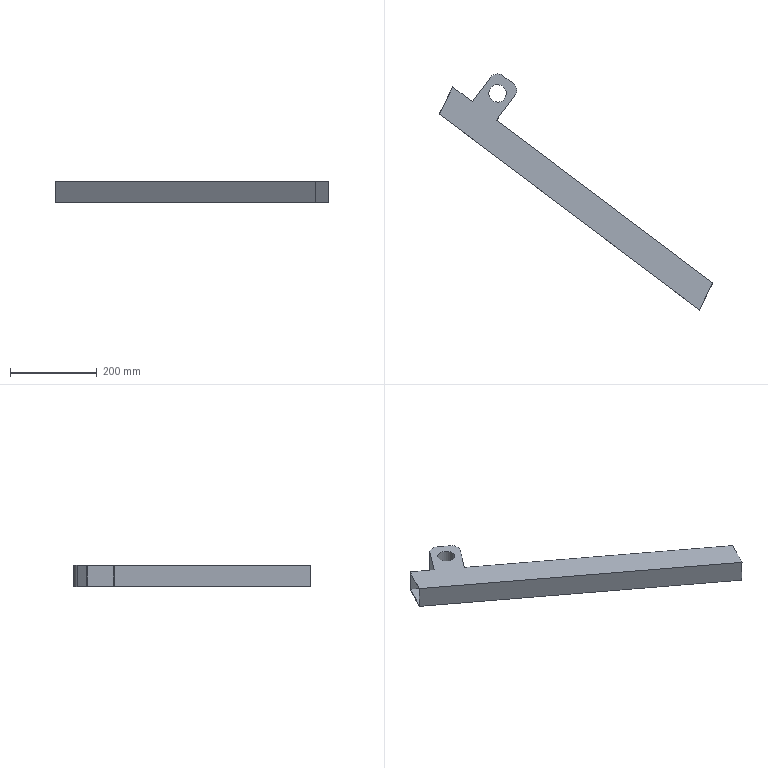Component | SolidWorks | FrameAssemblyDrawing11111-1_Part11-2 | 1 solid | 18 faces | box 629.99 x 543.02 x 50 mm | volume 587870 mm3 | plane 14 | cylinder 4 | commonest cylinder face diameters 40 x4
build123d program:
from build123d import *

# Parameters (mm, degrees)
BOSS_EXTRUDE1_DEPTH = 50
SHELL1_T            = -2
SKETCH2_R           = 20
BOSS_EXTRUDE2_DEPTH = 50


with BuildPart() as part:
    # Sketch1 → Boss-Extrude1 (new body)
    with BuildSketch(Plane.XY):
        Polygon((-43.98, -21.617), (705.02, -21.617), (692.745, 47.298), (-56.255, 47.298), align=None)
    extrude(amount=BOSS_EXTRUDE1_DEPTH)

    # Shell1
    shell1_openings = [part.faces().sort_by_distance(p)[0] for p in [
        (698.882, 12.841, 25),
        (-50.118, 12.841, 25),
    ]]
    offset(amount=SHELL1_T, openings=shell1_openings, kind=Kind.INTERSECTION)

    # Sketch2 → Boss-Extrude2 (add)
    with BuildSketch(Plane.XY.offset(50)):
        with BuildLine():
            Line((0, 47.298), (70, 47.298))
            Line((70, 47.298), (70, 117.298))
            ThreePointArc((70, 117.298), (64.142, 131.44), (50, 137.298))
            Line((50, 137.298), (20, 137.298))
            ThreePointArc((20, 137.298), (5.858, 131.44), (0, 117.298))
            Line((0, 117.298), (0, 47.298))
        make_face()
        with Locations((35, 97.298)):
            Circle(SKETCH2_R, mode=Mode.SUBTRACT)
    extrude(amount=-BOSS_EXTRUDE2_DEPTH)


solid = part.part

# Placed as in the assembly
solid = solid.moved(Location((-325.695, -673.671, 1035.971), (0, 0, -36.979)))
STEP:
#1=COLOUR_RGB('',0.7922,0.8196,0.9333);
#2=FILL_AREA_STYLE_COLOUR('',#1);
#3=FILL_AREA_STYLE('',(#2));
#4=SURFACE_STYLE_FILL_AREA(#3);
#5=SURFACE_SIDE_STYLE('',(#4));
#6=SURFACE_STYLE_USAGE(.BOTH.,#5);
#7=PRESENTATION_STYLE_ASSIGNMENT((#6));
#8=CARTESIAN_POINT('',(-10.047,-23.818,40.786));
#9=VERTEX_POINT('',#8);
#10=CARTESIAN_POINT('',(-8.789,-24.765,40.786));
#11=VERTEX_POINT('',#10);
#12=CARTESIAN_POINT('',(-9.418,-24.291,40.786));
#13=DIRECTION('',(-0.,-0.,1.));
#14=DIRECTION('',(0.7989,-0.6015,-0.));
#15=AXIS2_PLACEMENT_3D('',#12,#13,#14);
#16=CIRCLE('',#15,0.7874);
#17=EDGE_CURVE('',#9,#11,#16,.T.);
#18=ORIENTED_EDGE('',*,*,#17,.F.);
#19=CARTESIAN_POINT('',(-10.047,-23.818,42.755));
#20=VERTEX_POINT('',#19);
#21=CARTESIAN_POINT('',(-10.047,-23.818,40.786));
#22=DIRECTION('',(-0.,-0.,1.));
#23=VECTOR('',#22,39.37);
#24=LINE('',#21,#23);
#25=EDGE_CURVE('',#9,#20,#24,.T.);
#26=ORIENTED_EDGE('',*,*,#25,.T.);
#27=CARTESIAN_POINT('',(-8.789,-24.765,42.755));
#28=VERTEX_POINT('',#27);
#29=CARTESIAN_POINT('',(-9.418,-24.291,42.755));
#30=DIRECTION('',(-0.,-0.,1.));
#31=DIRECTION('',(0.7989,-0.6015,-0.));
#32=AXIS2_PLACEMENT_3D('',#29,#30,#31);
#33=CIRCLE('',#32,0.7874);
#34=EDGE_CURVE('',#20,#28,#33,.T.);
#35=ORIENTED_EDGE('',*,*,#34,.T.);
#36=CARTESIAN_POINT('',(-8.789,-24.765,40.786));
#37=DIRECTION('',(-0.,-0.,1.));
#38=VECTOR('',#37,39.37);
#39=LINE('',#36,#38);
#40=EDGE_CURVE('',#11,#28,#39,.T.);
#41=ORIENTED_EDGE('',*,*,#40,.F.);
#42=EDGE_LOOP('',(#18,#26,#35,#41));
#43=FACE_OUTER_BOUND('',#42,.T.);
#44=CARTESIAN_POINT('',(-9.418,-24.291,40.786));
#45=DIRECTION('',(-0.,-0.,1.));
#46=DIRECTION('',(0.7989,-0.6015,-0.));
#47=AXIS2_PLACEMENT_3D('',#44,#45,#46);
#48=CYLINDRICAL_SURFACE('',#47,0.7874);
#49=ADVANCED_FACE('',(#43),#48,.F.);
#50=CARTESIAN_POINT('',(-11.703,-25.035,40.786));
#51=VERTEX_POINT('',#50);
#52=CARTESIAN_POINT('',(-11.703,-25.035,42.755));
#53=VERTEX_POINT('',#52);
#54=CARTESIAN_POINT('',(-11.703,-25.035,40.786));
#55=DIRECTION('',(-0.,-0.,1.));
#56=VECTOR('',#55,39.37);
#57=LINE('',#54,#56);
#58=EDGE_CURVE('',#51,#53,#57,.T.);
#59=ORIENTED_EDGE('',*,*,#58,.F.);
#60=CARTESIAN_POINT('',(-13.472,-23.703,40.786));
#61=VERTEX_POINT('',#60);
#62=CARTESIAN_POINT('',(10.085,-41.44,40.786));
#63=DIRECTION('',(-0.7989,0.6015,0.));
#64=VECTOR('',#63,39.37);
#65=LINE('',#62,#64);
#66=EDGE_CURVE('',#51,#61,#65,.T.);
#67=ORIENTED_EDGE('',*,*,#66,.T.);
#68=CARTESIAN_POINT('',(-13.472,-23.703,42.755));
#69=VERTEX_POINT('',#68);
#70=CARTESIAN_POINT('',(-13.472,-23.703,42.755));
#71=DIRECTION('',(0.,0.,-1.));
#72=VECTOR('',#71,39.37);
#73=LINE('',#70,#72);
#74=EDGE_CURVE('',#69,#61,#73,.T.);
#75=ORIENTED_EDGE('',*,*,#74,.F.);
#76=CARTESIAN_POINT('',(10.085,-41.44,42.755));
#77=DIRECTION('',(-0.7989,0.6015,0.));
#78=VECTOR('',#77,39.37);
#79=LINE('',#76,#78);
#80=EDGE_CURVE('',#53,#69,#79,.T.);
#81=ORIENTED_EDGE('',*,*,#80,.F.);
#82=EDGE_LOOP('',(#59,#67,#75,#81));
#83=FACE_OUTER_BOUND('',#82,.T.);
#84=CARTESIAN_POINT('',(10.085,-41.44,42.755));
#85=DIRECTION('',(-0.6015,-0.7989,-0.));
#86=DIRECTION('',(0.,0.,-1.));
#87=AXIS2_PLACEMENT_3D('',#84,#85,#86);
#88=PLANE('',#87);
#89=ADVANCED_FACE('',(#83),#88,.F.);
#90=CARTESIAN_POINT('',(-14.718,-26.161,40.786));
#91=VERTEX_POINT('',#90);
#92=CARTESIAN_POINT('',(-14.718,-26.161,40.786));
#93=DIRECTION('',(-0.4521,-0.892,-0.));
#94=VECTOR('',#93,39.37);
#95=LINE('',#92,#94);
#96=EDGE_CURVE('',#61,#91,#95,.T.);
#97=ORIENTED_EDGE('',*,*,#96,.T.);
#98=CARTESIAN_POINT('',(-14.718,-26.161,42.755));
#99=VERTEX_POINT('',#98);
#100=CARTESIAN_POINT('',(-14.718,-26.161,42.755));
#101=DIRECTION('',(0.,0.,-1.));
#102=VECTOR('',#101,39.37);
#103=LINE('',#100,#102);
#104=EDGE_CURVE('',#99,#91,#103,.T.);
#105=ORIENTED_EDGE('',*,*,#104,.F.);
#106=CARTESIAN_POINT('',(-14.718,-26.161,42.755));
#107=DIRECTION('',(-0.4521,-0.892,-0.));
#108=VECTOR('',#107,39.37);
#109=LINE('',#106,#108);
#110=EDGE_CURVE('',#69,#99,#109,.T.);
#111=ORIENTED_EDGE('',*,*,#110,.F.);
#112=ORIENTED_EDGE('',*,*,#74,.T.);
#113=EDGE_LOOP('',(#97,#105,#111,#112));
#114=FACE_OUTER_BOUND('',#113,.T.);
#115=CARTESIAN_POINT('',(-13.508,-23.774,40.865));
#116=VERTEX_POINT('',#115);
#117=CARTESIAN_POINT('',(-14.682,-26.089,40.865));
#118=VERTEX_POINT('',#117);
#119=CARTESIAN_POINT('',(-14.718,-26.161,40.865));
#120=DIRECTION('',(-0.4521,-0.892,-0.));
#121=VECTOR('',#120,39.37);
#122=LINE('',#119,#121);
#123=EDGE_CURVE('',#116,#118,#122,.T.);
#124=ORIENTED_EDGE('',*,*,#123,.F.);
#125=CARTESIAN_POINT('',(-13.508,-23.774,42.676));
#126=VERTEX_POINT('',#125);
#127=CARTESIAN_POINT('',(-13.508,-23.774,42.755));
#128=DIRECTION('',(0.,0.,-1.));
#129=VECTOR('',#128,39.37);
#130=LINE('',#127,#129);
#131=EDGE_CURVE('',#126,#116,#130,.T.);
#132=ORIENTED_EDGE('',*,*,#131,.F.);
#133=CARTESIAN_POINT('',(-14.682,-26.089,42.676));
#134=VERTEX_POINT('',#133);
#135=CARTESIAN_POINT('',(-14.718,-26.161,42.676));
#136=DIRECTION('',(-0.4521,-0.892,-0.));
#137=VECTOR('',#136,39.37);
#138=LINE('',#135,#137);
#139=EDGE_CURVE('',#126,#134,#138,.T.);
#140=ORIENTED_EDGE('',*,*,#139,.T.);
#141=CARTESIAN_POINT('',(-14.682,-26.089,42.755));
#142=DIRECTION('',(0.,0.,-1.));
#143=VECTOR('',#142,39.37);
#144=LINE('',#141,#143);
#145=EDGE_CURVE('',#134,#118,#144,.T.);
#146=ORIENTED_EDGE('',*,*,#145,.T.);
#147=EDGE_LOOP('',(#124,#132,#140,#146));
#148=FACE_BOUND('',#147,.T.);
#149=CARTESIAN_POINT('',(-14.718,-26.161,42.755));
#150=DIRECTION('',(0.892,-0.4521,-0.));
#151=DIRECTION('',(0.4521,0.892,0.));
#152=AXIS2_PLACEMENT_3D('',#149,#150,#151);
#153=PLANE('',#152);
#154=ADVANCED_FACE('',(#114,#148),#153,.F.);
#155=CARTESIAN_POINT('',(8.839,-43.898,40.786));
#156=VERTEX_POINT('',#155);
#157=CARTESIAN_POINT('',(10.085,-41.44,40.786));
#158=VERTEX_POINT('',#157);
#159=CARTESIAN_POINT('',(8.839,-43.898,40.786));
#160=DIRECTION('',(0.4521,0.892,0.));
#161=VECTOR('',#160,39.37);
#162=LINE('',#159,#161);
#163=EDGE_CURVE('',#156,#158,#162,.T.);
#164=ORIENTED_EDGE('',*,*,#163,.T.);
#165=CARTESIAN_POINT('',(10.085,-41.44,42.755));
#166=VERTEX_POINT('',#165);
#167=CARTESIAN_POINT('',(10.085,-41.44,42.755));
#168=DIRECTION('',(0.,0.,-1.));
#169=VECTOR('',#168,39.37);
#170=LINE('',#167,#169);
#171=EDGE_CURVE('',#166,#158,#170,.T.);
#172=ORIENTED_EDGE('',*,*,#171,.F.);
#173=CARTESIAN_POINT('',(8.839,-43.898,42.755));
#174=VERTEX_POINT('',#173);
#175=CARTESIAN_POINT('',(8.839,-43.898,42.755));
#176=DIRECTION('',(0.4521,0.892,0.));
#177=VECTOR('',#176,39.37);
#178=LINE('',#175,#177);
#179=EDGE_CURVE('',#174,#166,#178,.T.);
#180=ORIENTED_EDGE('',*,*,#179,.F.);
#181=CARTESIAN_POINT('',(8.839,-43.898,42.755));
#182=DIRECTION('',(0.,0.,-1.));
#183=VECTOR('',#182,39.37);
#184=LINE('',#181,#183);
#185=EDGE_CURVE('',#174,#156,#184,.T.);
#186=ORIENTED_EDGE('',*,*,#185,.T.);
#187=EDGE_LOOP('',(#164,#172,#180,#186));
#188=FACE_OUTER_BOUND('',#187,.T.);
#189=CARTESIAN_POINT('',(8.875,-43.827,40.865));
#190=VERTEX_POINT('',#189);
#191=CARTESIAN_POINT('',(10.049,-41.512,40.865));
#192=VERTEX_POINT('',#191);
#193=CARTESIAN_POINT('',(8.839,-43.898,40.865));
#194=DIRECTION('',(0.4521,0.892,0.));
#195=VECTOR('',#194,39.37);
#196=LINE('',#193,#195);
#197=EDGE_CURVE('',#190,#192,#196,.T.);
#198=ORIENTED_EDGE('',*,*,#197,.F.);
#199=CARTESIAN_POINT('',(8.875,-43.827,42.676));
#200=VERTEX_POINT('',#199);
#201=CARTESIAN_POINT('',(8.875,-43.827,42.755));
#202=DIRECTION('',(0.,0.,-1.));
#203=VECTOR('',#202,39.37);
#204=LINE('',#201,#203);
#205=EDGE_CURVE('',#200,#190,#204,.T.);
#206=ORIENTED_EDGE('',*,*,#205,.F.);
#207=CARTESIAN_POINT('',(10.049,-41.512,42.676));
#208=VERTEX_POINT('',#207);
#209=CARTESIAN_POINT('',(8.839,-43.898,42.676));
#210=DIRECTION('',(0.4521,0.892,0.));
#211=VECTOR('',#210,39.37);
#212=LINE('',#209,#211);
#213=EDGE_CURVE('',#200,#208,#212,.T.);
#214=ORIENTED_EDGE('',*,*,#213,.T.);
#215=CARTESIAN_POINT('',(10.049,-41.512,42.755));
#216=DIRECTION('',(0.,0.,-1.));
#217=VECTOR('',#216,39.37);
#218=LINE('',#215,#217);
#219=EDGE_CURVE('',#208,#192,#218,.T.);
#220=ORIENTED_EDGE('',*,*,#219,.T.);
#221=EDGE_LOOP('',(#198,#206,#214,#220));
#222=FACE_BOUND('',#221,.T.);
#223=CARTESIAN_POINT('',(8.839,-43.898,42.755));
#224=DIRECTION('',(-0.892,0.4521,0.));
#225=DIRECTION('',(-0.4521,-0.892,-0.));
#226=AXIS2_PLACEMENT_3D('',#223,#224,#225);
#227=PLANE('',#226);
#228=ADVANCED_FACE('',(#188,#222),#227,.F.);
#229=CARTESIAN_POINT('',(-14.718,-26.161,40.786));
#230=DIRECTION('',(0.7989,-0.6015,-0.));
#231=VECTOR('',#230,39.37);
#232=LINE('',#229,#231);
#233=EDGE_CURVE('',#91,#156,#232,.T.);
#234=ORIENTED_EDGE('',*,*,#233,.T.);
#235=ORIENTED_EDGE('',*,*,#185,.F.);
#236=CARTESIAN_POINT('',(-14.718,-26.161,42.755));
#237=DIRECTION('',(0.7989,-0.6015,-0.));
#238=VECTOR('',#237,39.37);
#239=LINE('',#236,#238);
#240=EDGE_CURVE('',#99,#174,#239,.T.);
#241=ORIENTED_EDGE('',*,*,#240,.F.);
#242=ORIENTED_EDGE('',*,*,#104,.T.);
#243=EDGE_LOOP('',(#234,#235,#241,#242));
#244=FACE_OUTER_BOUND('',#243,.T.);
#245=CARTESIAN_POINT('',(-14.718,-26.161,42.755));
#246=DIRECTION('',(0.6015,0.7989,0.));
#247=DIRECTION('',(-0.,-0.,1.));
#248=AXIS2_PLACEMENT_3D('',#245,#246,#247);
#249=PLANE('',#248);
#250=ADVANCED_FACE('',(#244),#249,.F.);
#251=CARTESIAN_POINT('',(-9.501,-26.693,40.786));
#252=VERTEX_POINT('',#251);
#253=CARTESIAN_POINT('',(10.085,-41.44,40.786));
#254=DIRECTION('',(-0.7989,0.6015,0.));
#255=VECTOR('',#254,39.37);
#256=LINE('',#253,#255);
#257=EDGE_CURVE('',#158,#252,#256,.T.);
#258=ORIENTED_EDGE('',*,*,#257,.T.);
#259=CARTESIAN_POINT('',(-9.501,-26.693,42.755));
#260=VERTEX_POINT('',#259);
#261=CARTESIAN_POINT('',(-9.501,-26.693,40.786));
#262=DIRECTION('',(-0.,-0.,1.));
#263=VECTOR('',#262,39.37);
#264=LINE('',#261,#263);
#265=EDGE_CURVE('',#252,#260,#264,.T.);
#266=ORIENTED_EDGE('',*,*,#265,.T.);
#267=CARTESIAN_POINT('',(10.085,-41.44,42.755));
#268=DIRECTION('',(-0.7989,0.6015,0.));
#269=VECTOR('',#268,39.37);
#270=LINE('',#267,#269);
#271=EDGE_CURVE('',#166,#260,#270,.T.);
#272=ORIENTED_EDGE('',*,*,#271,.F.);
#273=ORIENTED_EDGE('',*,*,#171,.T.);
#274=EDGE_LOOP('',(#258,#266,#272,#273));
#275=FACE_OUTER_BOUND('',#274,.T.);
#276=CARTESIAN_POINT('',(10.085,-41.44,42.755));
#277=DIRECTION('',(-0.6015,-0.7989,-0.));
#278=DIRECTION('',(0.,0.,-1.));
#279=AXIS2_PLACEMENT_3D('',#276,#277,#278);
#280=PLANE('',#279);
#281=ADVANCED_FACE('',(#275),#280,.F.);
#282=ORIENTED_EDGE('',*,*,#110,.T.);
#283=ORIENTED_EDGE('',*,*,#240,.T.);
#284=ORIENTED_EDGE('',*,*,#179,.T.);
#285=ORIENTED_EDGE('',*,*,#271,.T.);
#286=CARTESIAN_POINT('',(-7.843,-24.491,42.755));
#287=VERTEX_POINT('',#286);
#288=CARTESIAN_POINT('',(-9.501,-26.693,42.755));
#289=DIRECTION('',(0.6015,0.7989,0.));
#290=VECTOR('',#289,39.37);
#291=LINE('',#288,#290);
#292=EDGE_CURVE('',#260,#287,#291,.T.);
#293=ORIENTED_EDGE('',*,*,#292,.T.);
#294=CARTESIAN_POINT('',(-7.999,-23.388,42.755));
#295=VERTEX_POINT('',#294);
#296=CARTESIAN_POINT('',(-8.472,-24.017,42.755));
#297=DIRECTION('',(-0.,-0.,1.));
#298=DIRECTION('',(0.7989,-0.6015,-0.));
#299=AXIS2_PLACEMENT_3D('',#296,#297,#298);
#300=CIRCLE('',#299,0.7874);
#301=EDGE_CURVE('',#287,#295,#300,.T.);
#302=ORIENTED_EDGE('',*,*,#301,.T.);
#303=CARTESIAN_POINT('',(-8.942,-22.678,42.755));
#304=VERTEX_POINT('',#303);
#305=CARTESIAN_POINT('',(-8.942,-22.678,42.755));
#306=DIRECTION('',(-0.7989,0.6015,0.));
#307=VECTOR('',#306,39.37);
#308=LINE('',#305,#307);
#309=EDGE_CURVE('',#295,#304,#308,.T.);
#310=ORIENTED_EDGE('',*,*,#309,.T.);
#311=CARTESIAN_POINT('',(-10.045,-22.833,42.755));
#312=VERTEX_POINT('',#311);
#313=CARTESIAN_POINT('',(-9.416,-23.307,42.755));
#314=DIRECTION('',(-0.,-0.,1.));
#315=DIRECTION('',(0.7989,-0.6015,-0.));
#316=AXIS2_PLACEMENT_3D('',#313,#314,#315);
#317=CIRCLE('',#316,0.7874);
#318=EDGE_CURVE('',#304,#312,#317,.T.);
#319=ORIENTED_EDGE('',*,*,#318,.T.);
#320=CARTESIAN_POINT('',(-11.703,-25.035,42.755));
#321=DIRECTION('',(-0.6015,-0.7989,-0.));
#322=VECTOR('',#321,39.37);
#323=LINE('',#320,#322);
#324=EDGE_CURVE('',#312,#53,#323,.T.);
#325=ORIENTED_EDGE('',*,*,#324,.T.);
#326=ORIENTED_EDGE('',*,*,#80,.T.);
#327=EDGE_LOOP('',(#282,#283,#284,#285,#293,#302,#310,#319,#325,#326));
#328=FACE_OUTER_BOUND('',#327,.T.);
#329=CARTESIAN_POINT('',(-9.418,-24.291,42.755));
#330=DIRECTION('',(-0.,-0.,1.));
#331=DIRECTION('',(0.7989,-0.6015,-0.));
#332=AXIS2_PLACEMENT_3D('',#329,#330,#331);
#333=CIRCLE('',#332,0.7874);
#334=EDGE_CURVE('',#28,#20,#333,.T.);
#335=ORIENTED_EDGE('',*,*,#334,.F.);
#336=ORIENTED_EDGE('',*,*,#34,.F.);
#337=EDGE_LOOP('',(#335,#336));
#338=FACE_BOUND('',#337,.T.);
#339=CARTESIAN_POINT('',(-12.823,-26.522,42.755));
#340=DIRECTION('',(-0.,-0.,1.));
#341=DIRECTION('',(0.7989,-0.6015,-0.));
#342=AXIS2_PLACEMENT_3D('',#339,#340,#341);
#343=PLANE('',#342);
#344=ADVANCED_FACE('',(#328,#338),#343,.T.);
#345=ORIENTED_EDGE('',*,*,#96,.F.);
#346=ORIENTED_EDGE('',*,*,#66,.F.);
#347=CARTESIAN_POINT('',(-10.045,-22.833,40.786));
#348=VERTEX_POINT('',#347);
#349=CARTESIAN_POINT('',(-11.703,-25.035,40.786));
#350=DIRECTION('',(-0.6015,-0.7989,-0.));
#351=VECTOR('',#350,39.37);
#352=LINE('',#349,#351);
#353=EDGE_CURVE('',#348,#51,#352,.T.);
#354=ORIENTED_EDGE('',*,*,#353,.F.);
#355=CARTESIAN_POINT('',(-8.942,-22.678,40.786));
#356=VERTEX_POINT('',#355);
#357=CARTESIAN_POINT('',(-9.416,-23.307,40.786));
#358=DIRECTION('',(-0.,-0.,1.));
#359=DIRECTION('',(0.7989,-0.6015,-0.));
#360=AXIS2_PLACEMENT_3D('',#357,#358,#359);
#361=CIRCLE('',#360,0.7874);
#362=EDGE_CURVE('',#356,#348,#361,.T.);
#363=ORIENTED_EDGE('',*,*,#362,.F.);
#364=CARTESIAN_POINT('',(-7.999,-23.388,40.786));
#365=VERTEX_POINT('',#364);
#366=CARTESIAN_POINT('',(-8.942,-22.678,40.786));
#367=DIRECTION('',(-0.7989,0.6015,0.));
#368=VECTOR('',#367,39.37);
#369=LINE('',#366,#368);
#370=EDGE_CURVE('',#365,#356,#369,.T.);
#371=ORIENTED_EDGE('',*,*,#370,.F.);
#372=CARTESIAN_POINT('',(-7.843,-24.491,40.786));
#373=VERTEX_POINT('',#372);
#374=CARTESIAN_POINT('',(-8.472,-24.017,40.786));
#375=DIRECTION('',(-0.,-0.,1.));
#376=DIRECTION('',(0.7989,-0.6015,-0.));
#377=AXIS2_PLACEMENT_3D('',#374,#375,#376);
#378=CIRCLE('',#377,0.7874);
#379=EDGE_CURVE('',#373,#365,#378,.T.);
#380=ORIENTED_EDGE('',*,*,#379,.F.);
#381=CARTESIAN_POINT('',(-9.501,-26.693,40.786));
#382=DIRECTION('',(0.6015,0.7989,0.));
#383=VECTOR('',#382,39.37);
#384=LINE('',#381,#383);
#385=EDGE_CURVE('',#252,#373,#384,.T.);
#386=ORIENTED_EDGE('',*,*,#385,.F.);
#387=ORIENTED_EDGE('',*,*,#257,.F.);
#388=ORIENTED_EDGE('',*,*,#163,.F.);
#389=ORIENTED_EDGE('',*,*,#233,.F.);
#390=EDGE_LOOP('',(#345,#346,#354,#363,#371,#380,#386,#387,#388,#389));
#391=FACE_OUTER_BOUND('',#390,.T.);
#392=CARTESIAN_POINT('',(-9.418,-24.291,40.786));
#393=DIRECTION('',(-0.,-0.,1.));
#394=DIRECTION('',(0.7989,-0.6015,-0.));
#395=AXIS2_PLACEMENT_3D('',#392,#393,#394);
#396=CIRCLE('',#395,0.7874);
#397=EDGE_CURVE('',#11,#9,#396,.T.);
#398=ORIENTED_EDGE('',*,*,#397,.T.);
#399=ORIENTED_EDGE('',*,*,#17,.T.);
#400=EDGE_LOOP('',(#398,#399));
#401=FACE_BOUND('',#400,.T.);
#402=CARTESIAN_POINT('',(-12.823,-26.522,40.786));
#403=DIRECTION('',(-0.,-0.,1.));
#404=DIRECTION('',(0.7989,-0.6015,-0.));
#405=AXIS2_PLACEMENT_3D('',#402,#403,#404);
#406=PLANE('',#405);
#407=ADVANCED_FACE('',(#391,#401),#406,.F.);
#408=CARTESIAN_POINT('',(-14.67,-26.098,40.865));
#409=DIRECTION('',(0.7989,-0.6015,-0.));
#410=VECTOR('',#409,39.37);
#411=LINE('',#408,#410);
#412=EDGE_CURVE('',#118,#190,#411,.T.);
#413=ORIENTED_EDGE('',*,*,#412,.F.);
#414=ORIENTED_EDGE('',*,*,#145,.F.);
#415=CARTESIAN_POINT('',(-14.67,-26.098,42.676));
#416=DIRECTION('',(0.7989,-0.6015,-0.));
#417=VECTOR('',#416,39.37);
#418=LINE('',#415,#417);
#419=EDGE_CURVE('',#134,#200,#418,.T.);
#420=ORIENTED_EDGE('',*,*,#419,.T.);
#421=ORIENTED_EDGE('',*,*,#205,.T.);
#422=EDGE_LOOP('',(#413,#414,#420,#421));
#423=FACE_OUTER_BOUND('',#422,.T.);
#424=CARTESIAN_POINT('',(-14.67,-26.098,42.755));
#425=DIRECTION('',(0.6015,0.7989,0.));
#426=DIRECTION('',(-0.,-0.,1.));
#427=AXIS2_PLACEMENT_3D('',#424,#425,#426);
#428=PLANE('',#427);
#429=ADVANCED_FACE('',(#423),#428,.T.);
#430=CARTESIAN_POINT('',(10.038,-41.503,40.865));
#431=DIRECTION('',(-0.7989,0.6015,0.));
#432=VECTOR('',#431,39.37);
#433=LINE('',#430,#432);
#434=EDGE_CURVE('',#192,#116,#433,.T.);
#435=ORIENTED_EDGE('',*,*,#434,.F.);
#436=ORIENTED_EDGE('',*,*,#219,.F.);
#437=CARTESIAN_POINT('',(10.038,-41.503,42.676));
#438=DIRECTION('',(-0.7989,0.6015,0.));
#439=VECTOR('',#438,39.37);
#440=LINE('',#437,#439);
#441=EDGE_CURVE('',#208,#126,#440,.T.);
#442=ORIENTED_EDGE('',*,*,#441,.T.);
#443=ORIENTED_EDGE('',*,*,#131,.T.);
#444=EDGE_LOOP('',(#435,#436,#442,#443));
#445=FACE_OUTER_BOUND('',#444,.T.);
#446=CARTESIAN_POINT('',(10.038,-41.503,42.755));
#447=DIRECTION('',(-0.6015,-0.7989,-0.));
#448=DIRECTION('',(0.,0.,-1.));
#449=AXIS2_PLACEMENT_3D('',#446,#447,#448);
#450=PLANE('',#449);
#451=ADVANCED_FACE('',(#445),#450,.T.);
#452=ORIENTED_EDGE('',*,*,#139,.F.);
#453=ORIENTED_EDGE('',*,*,#441,.F.);
#454=ORIENTED_EDGE('',*,*,#213,.F.);
#455=ORIENTED_EDGE('',*,*,#419,.F.);
#456=EDGE_LOOP('',(#452,#453,#454,#455));
#457=FACE_OUTER_BOUND('',#456,.T.);
#458=CARTESIAN_POINT('',(-12.823,-26.522,42.676));
#459=DIRECTION('',(-0.,-0.,1.));
#460=DIRECTION('',(0.7989,-0.6015,-0.));
#461=AXIS2_PLACEMENT_3D('',#458,#459,#460);
#462=PLANE('',#461);
#463=ADVANCED_FACE('',(#457),#462,.F.);
#464=ORIENTED_EDGE('',*,*,#123,.T.);
#465=ORIENTED_EDGE('',*,*,#412,.T.);
#466=ORIENTED_EDGE('',*,*,#197,.T.);
#467=ORIENTED_EDGE('',*,*,#434,.T.);
#468=EDGE_LOOP('',(#464,#465,#466,#467));
#469=FACE_OUTER_BOUND('',#468,.T.);
#470=CARTESIAN_POINT('',(-12.823,-26.522,40.865));
#471=DIRECTION('',(-0.,-0.,1.));
#472=DIRECTION('',(0.7989,-0.6015,-0.));
#473=AXIS2_PLACEMENT_3D('',#470,#471,#472);
#474=PLANE('',#473);
#475=ADVANCED_FACE('',(#469),#474,.T.);
#476=ORIENTED_EDGE('',*,*,#324,.F.);
#477=CARTESIAN_POINT('',(-10.045,-22.833,40.786));
#478=DIRECTION('',(-0.,-0.,1.));
#479=VECTOR('',#478,39.37);
#480=LINE('',#477,#479);
#481=EDGE_CURVE('',#348,#312,#480,.T.);
#482=ORIENTED_EDGE('',*,*,#481,.F.);
#483=ORIENTED_EDGE('',*,*,#353,.T.);
#484=ORIENTED_EDGE('',*,*,#58,.T.);
#485=EDGE_LOOP('',(#476,#482,#483,#484));
#486=FACE_OUTER_BOUND('',#485,.T.);
#487=CARTESIAN_POINT('',(-11.703,-25.035,40.786));
#488=DIRECTION('',(-0.7989,0.6015,0.));
#489=DIRECTION('',(-0.,-0.,1.));
#490=AXIS2_PLACEMENT_3D('',#487,#488,#489);
#491=PLANE('',#490);
#492=ADVANCED_FACE('',(#486),#491,.T.);
#493=ORIENTED_EDGE('',*,*,#318,.F.);
#494=CARTESIAN_POINT('',(-8.942,-22.678,40.786));
#495=DIRECTION('',(-0.,-0.,1.));
#496=VECTOR('',#495,39.37);
#497=LINE('',#494,#496);
#498=EDGE_CURVE('',#356,#304,#497,.T.);
#499=ORIENTED_EDGE('',*,*,#498,.F.);
#500=ORIENTED_EDGE('',*,*,#362,.T.);
#501=ORIENTED_EDGE('',*,*,#481,.T.);
#502=EDGE_LOOP('',(#493,#499,#500,#501));
#503=FACE_OUTER_BOUND('',#502,.T.);
#504=CARTESIAN_POINT('',(-9.416,-23.307,40.786));
#505=DIRECTION('',(-0.,-0.,1.));
#506=DIRECTION('',(0.7989,-0.6015,-0.));
#507=AXIS2_PLACEMENT_3D('',#504,#505,#506);
#508=CYLINDRICAL_SURFACE('',#507,0.7874);
#509=ADVANCED_FACE('',(#503),#508,.T.);
#510=ORIENTED_EDGE('',*,*,#309,.F.);
#511=CARTESIAN_POINT('',(-7.999,-23.388,40.786));
#512=DIRECTION('',(-0.,-0.,1.));
#513=VECTOR('',#512,39.37);
#514=LINE('',#511,#513);
#515=EDGE_CURVE('',#365,#295,#514,.T.);
#516=ORIENTED_EDGE('',*,*,#515,.F.);
#517=ORIENTED_EDGE('',*,*,#370,.T.);
#518=ORIENTED_EDGE('',*,*,#498,.T.);
#519=EDGE_LOOP('',(#510,#516,#517,#518));
#520=FACE_OUTER_BOUND('',#519,.T.);
#521=CARTESIAN_POINT('',(-8.942,-22.678,40.786));
#522=DIRECTION('',(0.6015,0.7989,0.));
#523=DIRECTION('',(-0.,-0.,1.));
#524=AXIS2_PLACEMENT_3D('',#521,#522,#523);
#525=PLANE('',#524);
#526=ADVANCED_FACE('',(#520),#525,.T.);
#527=ORIENTED_EDGE('',*,*,#301,.F.);
#528=CARTESIAN_POINT('',(-7.843,-24.491,40.786));
#529=DIRECTION('',(-0.,-0.,1.));
#530=VECTOR('',#529,39.37);
#531=LINE('',#528,#530);
#532=EDGE_CURVE('',#373,#287,#531,.T.);
#533=ORIENTED_EDGE('',*,*,#532,.F.);
#534=ORIENTED_EDGE('',*,*,#379,.T.);
#535=ORIENTED_EDGE('',*,*,#515,.T.);
#536=EDGE_LOOP('',(#527,#533,#534,#535));
#537=FACE_OUTER_BOUND('',#536,.T.);
#538=CARTESIAN_POINT('',(-8.472,-24.017,40.786));
#539=DIRECTION('',(-0.,-0.,1.));
#540=DIRECTION('',(0.7989,-0.6015,-0.));
#541=AXIS2_PLACEMENT_3D('',#538,#539,#540);
#542=CYLINDRICAL_SURFACE('',#541,0.7874);
#543=ADVANCED_FACE('',(#537),#542,.T.);
#544=ORIENTED_EDGE('',*,*,#292,.F.);
#545=ORIENTED_EDGE('',*,*,#265,.F.);
#546=ORIENTED_EDGE('',*,*,#385,.T.);
#547=ORIENTED_EDGE('',*,*,#532,.T.);
#548=EDGE_LOOP('',(#544,#545,#546,#547));
#549=FACE_OUTER_BOUND('',#548,.T.);
#550=CARTESIAN_POINT('',(-9.501,-26.693,40.786));
#551=DIRECTION('',(0.7989,-0.6015,-0.));
#552=DIRECTION('',(0.,0.,-1.));
#553=AXIS2_PLACEMENT_3D('',#550,#551,#552);
#554=PLANE('',#553);
#555=ADVANCED_FACE('',(#549),#554,.T.);
#556=ORIENTED_EDGE('',*,*,#25,.F.);
#557=ORIENTED_EDGE('',*,*,#397,.F.);
#558=ORIENTED_EDGE('',*,*,#40,.T.);
#559=ORIENTED_EDGE('',*,*,#334,.T.);
#560=EDGE_LOOP('',(#556,#557,#558,#559));
#561=FACE_OUTER_BOUND('',#560,.T.);
#562=CARTESIAN_POINT('',(-9.418,-24.291,40.786));
#563=DIRECTION('',(-0.,-0.,1.));
#564=DIRECTION('',(0.7989,-0.6015,-0.));
#565=AXIS2_PLACEMENT_3D('',#562,#563,#564);
#566=CYLINDRICAL_SURFACE('',#565,0.7874);
#567=ADVANCED_FACE('',(#561),#566,.F.);
#568=CLOSED_SHELL('',(#49,#89,#154,#228,#250,#281,#344,#407,#429,#451,#463,#475,#492,#509,#526,#543,#555,#567));
#569=MANIFOLD_SOLID_BREP('',#568);
#570=STYLED_ITEM('',(#7),#569);
#571=(LENGTH_UNIT()NAMED_UNIT(*)SI_UNIT($,.METRE.));
#572=LENGTH_MEASURE_WITH_UNIT(LENGTH_MEASURE(0.0254),#571);
#573=DIMENSIONAL_EXPONENTS(1.,0.,0.,0.,0.,0.,0.);
#574=(CONVERSION_BASED_UNIT('',#572)LENGTH_UNIT()NAMED_UNIT(#573));
#575=UNCERTAINTY_MEASURE_WITH_UNIT(LENGTH_MEASURE(0.00001),#574,'','');
#576=(NAMED_UNIT(*)PLANE_ANGLE_UNIT()SI_UNIT($,.RADIAN.));
#577=(NAMED_UNIT(*)SI_UNIT($,.STERADIAN.)SOLID_ANGLE_UNIT());
#578=(GEOMETRIC_REPRESENTATION_CONTEXT(3)GLOBAL_UNCERTAINTY_ASSIGNED_CONTEXT((#575))GLOBAL_UNIT_ASSIGNED_CONTEXT((#574,#576,#577))REPRESENTATION_CONTEXT('',''));
#579=MECHANICAL_DESIGN_GEOMETRIC_PRESENTATION_REPRESENTATION('',(#570),#578);
#580=PRESENTATION_LAYER_ASSIGNMENT('','',(#570));
#581=CARTESIAN_POINT('',(0.,0.,0.));
#582=DIRECTION('',(0.,0.,1.));
#583=DIRECTION('',(1.,0.,0.));
#584=AXIS2_PLACEMENT_3D('',#581,#582,#583);
#585=(LENGTH_UNIT()NAMED_UNIT(*)SI_UNIT($,.METRE.));
#586=LENGTH_MEASURE_WITH_UNIT(LENGTH_MEASURE(0.0254),#585);
#587=DIMENSIONAL_EXPONENTS(1.,0.,0.,0.,0.,0.,0.);
#588=(CONVERSION_BASED_UNIT('',#586)LENGTH_UNIT()NAMED_UNIT(#587));
#589=UNCERTAINTY_MEASURE_WITH_UNIT(LENGTH_MEASURE(0.00001),#588,'','');
#590=(NAMED_UNIT(*)PLANE_ANGLE_UNIT()SI_UNIT($,.RADIAN.));
#591=(NAMED_UNIT(*)SI_UNIT($,.STERADIAN.)SOLID_ANGLE_UNIT());
#592=(GEOMETRIC_REPRESENTATION_CONTEXT(3)GLOBAL_UNCERTAINTY_ASSIGNED_CONTEXT((#589))GLOBAL_UNIT_ASSIGNED_CONTEXT((#588,#590,#591))REPRESENTATION_CONTEXT('',''));
#593=ADVANCED_BREP_SHAPE_REPRESENTATION('',(#569,#584),#592);